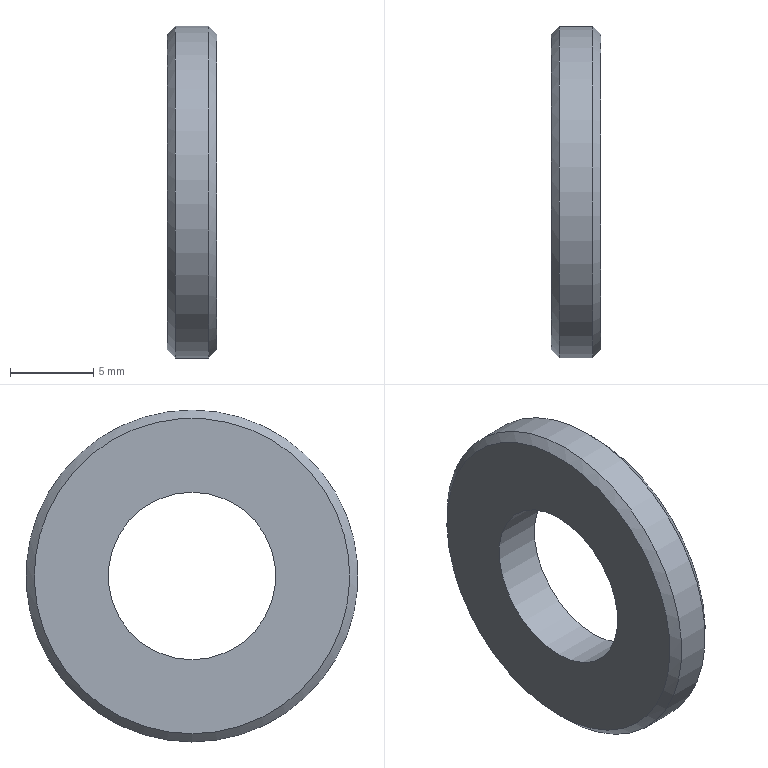Component | NX | 11_WASHER | 1 solid | 6 faces | box 3 x 20 x 20 mm | volume 687 mm3 | plane 2 | cylinder 2 | cone 2 | commonest cylinder face diameters 10.1 x1 20 x1
STEP:
#1=CARTESIAN_POINT('',(0.,0.,0.));
#2=DIRECTION('',(0.,0.,1.));
#3=DIRECTION('',(1.,0.,0.));
#4=AXIS2_PLACEMENT_3D('',#1,#2,#3);
#5=CARTESIAN_POINT('',(-0.,-0.,72.5));
#6=VERTEX_POINT('',#5);
#7=CARTESIAN_POINT('',(-0.,-0.,63.));
#8=DIRECTION('',(1.,0.,0.));
#9=DIRECTION('',(0.,0.,1.));
#10=AXIS2_PLACEMENT_3D('',#7,#8,#9);
#11=CIRCLE('',#10,9.5);
#12=CARTESIAN_POINT('',(-0.,-0.,73.));
#13=DIRECTION('',(-1.,0.,0.));
#14=DIRECTION('',(0.,0.,1.));
#15=AXIS2_PLACEMENT_3D('',#12,#13,#14);
#16=PLANE('',#15);
#17=CARTESIAN_POINT('',(-0.5,0.));
#18=CARTESIAN_POINT('',(-0.5,-16.454));
#19=CARTESIAN_POINT('',(-14.75,-8.227));
#20=CARTESIAN_POINT('',(-29.,-0.));
#21=CARTESIAN_POINT('',(-14.75,8.227));
#22=CARTESIAN_POINT('',(-0.5,16.454));
#23=CARTESIAN_POINT('',(-0.5,0.));
#24=(BOUNDED_CURVE()B_SPLINE_CURVE(2,(#17,#18,#19,#20,#21,#22,#23),.UNSPECIFIED.,.T.,.F.)B_SPLINE_CURVE_WITH_KNOTS((1,2,2,2,2,1),(-2.094,0.,2.094,4.189,6.283,8.378),.UNSPECIFIED.)CURVE()GEOMETRIC_REPRESENTATION_ITEM()RATIONAL_B_SPLINE_CURVE((1.,0.5,1.,0.5,1.,0.5,1.))REPRESENTATION_ITEM(''));
#25=(GEOMETRIC_REPRESENTATION_CONTEXT(2)PARAMETRIC_REPRESENTATION_CONTEXT()REPRESENTATION_CONTEXT('',''));
#26=DEFINITIONAL_REPRESENTATION('',(#24),#25);
#27=PCURVE('',#16,#26);
#28=CARTESIAN_POINT('',(-0.,-0.,63.));
#29=DIRECTION('',(-1.,0.,0.));
#30=DIRECTION('',(0.,0.,1.));
#31=AXIS2_PLACEMENT_3D('',#28,#29,#30);
#32=CONICAL_SURFACE('',#31,9.5,0.7854);
#33=CARTESIAN_POINT('',(6.283,0.));
#34=DIRECTION('',(-1.,0.));
#35=VECTOR('',#34,1.);
#36=LINE('',#33,#35);
#37=(GEOMETRIC_REPRESENTATION_CONTEXT(2)PARAMETRIC_REPRESENTATION_CONTEXT()REPRESENTATION_CONTEXT('',''));
#38=DEFINITIONAL_REPRESENTATION('',(#36),#37);
#39=PCURVE('',#32,#38);
#40=SURFACE_CURVE('',#11,(#27,#39),.PCURVE_S1.);
#41=EDGE_CURVE('',#6,#6,#40,.T.);
#42=ORIENTED_EDGE('',*,*,#41,.T.);
#43=EDGE_LOOP('',(#42));
#44=FACE_BOUND('',#43,.T.);
#45=CARTESIAN_POINT('',(0.,-0.,57.95));
#46=VERTEX_POINT('',#45);
#47=CARTESIAN_POINT('',(0.,-0.,63.));
#48=DIRECTION('',(1.,0.,0.));
#49=DIRECTION('',(0.,0.,-1.));
#50=AXIS2_PLACEMENT_3D('',#47,#48,#49);
#51=CIRCLE('',#50,5.05);
#52=CARTESIAN_POINT('',(-15.05,0.));
#53=CARTESIAN_POINT('',(-15.05,8.747));
#54=CARTESIAN_POINT('',(-7.475,4.373));
#55=CARTESIAN_POINT('',(0.1,0.));
#56=CARTESIAN_POINT('',(-7.475,-4.373));
#57=CARTESIAN_POINT('',(-15.05,-8.747));
#58=CARTESIAN_POINT('',(-15.05,0.));
#59=(BOUNDED_CURVE()B_SPLINE_CURVE(2,(#52,#53,#54,#55,#56,#57,#58),.UNSPECIFIED.,.T.,.F.)B_SPLINE_CURVE_WITH_KNOTS((1,2,2,2,2,1),(-2.094,0.,2.094,4.189,6.283,8.378),.UNSPECIFIED.)CURVE()GEOMETRIC_REPRESENTATION_ITEM()RATIONAL_B_SPLINE_CURVE((1.,0.5,1.,0.5,1.,0.5,1.))REPRESENTATION_ITEM(''));
#60=(GEOMETRIC_REPRESENTATION_CONTEXT(2)PARAMETRIC_REPRESENTATION_CONTEXT()REPRESENTATION_CONTEXT('',''));
#61=DEFINITIONAL_REPRESENTATION('',(#59),#60);
#62=PCURVE('',#16,#61);
#63=CARTESIAN_POINT('',(0.,-0.,63.));
#64=DIRECTION('',(1.,0.,0.));
#65=DIRECTION('',(0.,0.,-1.));
#66=AXIS2_PLACEMENT_3D('',#63,#64,#65);
#67=CYLINDRICAL_SURFACE('',#66,5.05);
#68=CARTESIAN_POINT('',(0.,0.));
#69=DIRECTION('',(1.,0.));
#70=VECTOR('',#69,1.);
#71=LINE('',#68,#70);
#72=(GEOMETRIC_REPRESENTATION_CONTEXT(2)PARAMETRIC_REPRESENTATION_CONTEXT()REPRESENTATION_CONTEXT('',''));
#73=DEFINITIONAL_REPRESENTATION('',(#71),#72);
#74=PCURVE('',#67,#73);
#75=SURFACE_CURVE('',#51,(#62,#74),.PCURVE_S1.);
#76=EDGE_CURVE('',#46,#46,#75,.T.);
#77=ORIENTED_EDGE('',*,*,#76,.F.);
#78=EDGE_LOOP('',(#77));
#79=FACE_BOUND('',#78,.T.);
#80=ADVANCED_FACE('',(#44,#79),#16,.F.);
#81=CARTESIAN_POINT('',(-3.,-0.,57.95));
#82=VERTEX_POINT('',#81);
#83=CARTESIAN_POINT('',(-3.,-0.,63.));
#84=DIRECTION('',(1.,0.,0.));
#85=DIRECTION('',(0.,0.,-1.));
#86=AXIS2_PLACEMENT_3D('',#83,#84,#85);
#87=CIRCLE('',#86,5.05);
#88=CARTESIAN_POINT('',(0.,-3.));
#89=DIRECTION('',(1.,0.));
#90=VECTOR('',#89,1.);
#91=LINE('',#88,#90);
#92=(GEOMETRIC_REPRESENTATION_CONTEXT(2)PARAMETRIC_REPRESENTATION_CONTEXT()REPRESENTATION_CONTEXT('',''));
#93=DEFINITIONAL_REPRESENTATION('',(#91),#92);
#94=PCURVE('',#67,#93);
#95=CARTESIAN_POINT('',(-3.,-0.,68.05));
#96=DIRECTION('',(1.,0.,0.));
#97=DIRECTION('',(0.,0.,-1.));
#98=AXIS2_PLACEMENT_3D('',#95,#96,#97);
#99=PLANE('',#98);
#100=CARTESIAN_POINT('',(5.05,0.));
#101=DIRECTION('',(1.,0.));
#102=AXIS2_PLACEMENT_2D('',#100,#101);
#103=CIRCLE('',#102,5.05);
#104=(GEOMETRIC_REPRESENTATION_CONTEXT(2)PARAMETRIC_REPRESENTATION_CONTEXT()REPRESENTATION_CONTEXT('',''));
#105=DEFINITIONAL_REPRESENTATION('',(#103),#104);
#106=PCURVE('',#99,#105);
#107=SURFACE_CURVE('',#87,(#94,#106),.PCURVE_S1.);
#108=EDGE_CURVE('',#82,#82,#107,.T.);
#109=ORIENTED_EDGE('',*,*,#108,.T.);
#110=CARTESIAN_POINT('',(-3.,-0.,57.95));
#111=CARTESIAN_POINT('',(0.,-0.,57.95));
#112=B_SPLINE_CURVE_WITH_KNOTS('',1,(#110,#111),.UNSPECIFIED.,.F.,.F.,(2,2),(-3.,0.),.PIECEWISE_BEZIER_KNOTS.);
#113=CARTESIAN_POINT('',(6.283,0.));
#114=DIRECTION('',(0.,1.));
#115=VECTOR('',#114,1.);
#116=LINE('',#113,#115);
#117=(GEOMETRIC_REPRESENTATION_CONTEXT(2)PARAMETRIC_REPRESENTATION_CONTEXT()REPRESENTATION_CONTEXT('',''));
#118=DEFINITIONAL_REPRESENTATION('',(#116),#117);
#119=PCURVE('',#67,#118);
#120=CARTESIAN_POINT('',(0.,0.));
#121=DIRECTION('',(0.,1.));
#122=VECTOR('',#121,1.);
#123=LINE('',#120,#122);
#124=(GEOMETRIC_REPRESENTATION_CONTEXT(2)PARAMETRIC_REPRESENTATION_CONTEXT()REPRESENTATION_CONTEXT('',''));
#125=DEFINITIONAL_REPRESENTATION('',(#123),#124);
#126=PCURVE('',#67,#125);
#127=SEAM_CURVE('',#112,(#119,#126),.PCURVE_S1.);
#128=EDGE_CURVE('',#82,#46,#127,.T.);
#129=ORIENTED_EDGE('',*,*,#128,.T.);
#130=ORIENTED_EDGE('',*,*,#76,.F.);
#131=ORIENTED_EDGE('',*,*,#128,.F.);
#132=EDGE_LOOP('',(#109,#129,#130,#131));
#133=FACE_BOUND('',#132,.F.);
#134=ADVANCED_FACE('',(#133),#67,.F.);
#135=CARTESIAN_POINT('',(-3.,-0.,53.5));
#136=VERTEX_POINT('',#135);
#137=CARTESIAN_POINT('',(-3.,-0.,63.));
#138=DIRECTION('',(-1.,0.,0.));
#139=DIRECTION('',(0.,0.,-1.));
#140=AXIS2_PLACEMENT_3D('',#137,#138,#139);
#141=CIRCLE('',#140,9.5);
#142=CARTESIAN_POINT('',(14.55,0.));
#143=CARTESIAN_POINT('',(14.55,-16.454));
#144=CARTESIAN_POINT('',(0.3,-8.227));
#145=CARTESIAN_POINT('',(-13.95,-0.));
#146=CARTESIAN_POINT('',(0.3,8.227));
#147=CARTESIAN_POINT('',(14.55,16.454));
#148=CARTESIAN_POINT('',(14.55,0.));
#149=(BOUNDED_CURVE()B_SPLINE_CURVE(2,(#142,#143,#144,#145,#146,#147,#148),.UNSPECIFIED.,.T.,.F.)B_SPLINE_CURVE_WITH_KNOTS((1,2,2,2,2,1),(-2.094,0.,2.094,4.189,6.283,8.378),.UNSPECIFIED.)CURVE()GEOMETRIC_REPRESENTATION_ITEM()RATIONAL_B_SPLINE_CURVE((1.,0.5,1.,0.5,1.,0.5,1.))REPRESENTATION_ITEM(''));
#150=(GEOMETRIC_REPRESENTATION_CONTEXT(2)PARAMETRIC_REPRESENTATION_CONTEXT()REPRESENTATION_CONTEXT('',''));
#151=DEFINITIONAL_REPRESENTATION('',(#149),#150);
#152=PCURVE('',#99,#151);
#153=CARTESIAN_POINT('',(-2.5,-0.,63.));
#154=DIRECTION('',(1.,0.,0.));
#155=DIRECTION('',(0.,0.,-1.));
#156=AXIS2_PLACEMENT_3D('',#153,#154,#155);
#157=CONICAL_SURFACE('',#156,10.,0.7854);
#158=CARTESIAN_POINT('',(6.283,-0.5));
#159=DIRECTION('',(-1.,0.));
#160=VECTOR('',#159,1.);
#161=LINE('',#158,#160);
#162=(GEOMETRIC_REPRESENTATION_CONTEXT(2)PARAMETRIC_REPRESENTATION_CONTEXT()REPRESENTATION_CONTEXT('',''));
#163=DEFINITIONAL_REPRESENTATION('',(#161),#162);
#164=PCURVE('',#157,#163);
#165=SURFACE_CURVE('',#141,(#152,#164),.PCURVE_S1.);
#166=EDGE_CURVE('',#136,#136,#165,.T.);
#167=ORIENTED_EDGE('',*,*,#166,.T.);
#168=EDGE_LOOP('',(#167));
#169=FACE_BOUND('',#168,.T.);
#170=ORIENTED_EDGE('',*,*,#108,.T.);
#171=EDGE_LOOP('',(#170));
#172=FACE_BOUND('',#171,.T.);
#173=ADVANCED_FACE('',(#169,#172),#99,.F.);
#174=CARTESIAN_POINT('',(-2.5,-0.,53.));
#175=VERTEX_POINT('',#174);
#176=CARTESIAN_POINT('',(-2.5,-0.,63.));
#177=DIRECTION('',(1.,0.,0.));
#178=DIRECTION('',(0.,0.,-1.));
#179=AXIS2_PLACEMENT_3D('',#176,#177,#178);
#180=CIRCLE('',#179,10.);
#181=CARTESIAN_POINT('',(0.,-0.,63.));
#182=DIRECTION('',(1.,0.,0.));
#183=DIRECTION('',(0.,0.,-1.));
#184=AXIS2_PLACEMENT_3D('',#181,#182,#183);
#185=CYLINDRICAL_SURFACE('',#184,10.);
#186=CARTESIAN_POINT('',(0.,-2.5));
#187=DIRECTION('',(1.,0.));
#188=VECTOR('',#187,1.);
#189=LINE('',#186,#188);
#190=(GEOMETRIC_REPRESENTATION_CONTEXT(2)PARAMETRIC_REPRESENTATION_CONTEXT()REPRESENTATION_CONTEXT('',''));
#191=DEFINITIONAL_REPRESENTATION('',(#189),#190);
#192=PCURVE('',#185,#191);
#193=CARTESIAN_POINT('',(0.,0.));
#194=DIRECTION('',(1.,0.));
#195=VECTOR('',#194,1.);
#196=LINE('',#193,#195);
#197=(GEOMETRIC_REPRESENTATION_CONTEXT(2)PARAMETRIC_REPRESENTATION_CONTEXT()REPRESENTATION_CONTEXT('',''));
#198=DEFINITIONAL_REPRESENTATION('',(#196),#197);
#199=PCURVE('',#157,#198);
#200=SURFACE_CURVE('',#180,(#192,#199),.PCURVE_S1.);
#201=EDGE_CURVE('',#175,#175,#200,.T.);
#202=ORIENTED_EDGE('',*,*,#201,.T.);
#203=CARTESIAN_POINT('',(-0.5,-0.,53.));
#204=VERTEX_POINT('',#203);
#205=CARTESIAN_POINT('',(-2.5,-0.,53.));
#206=CARTESIAN_POINT('',(-0.5,-0.,53.));
#207=B_SPLINE_CURVE_WITH_KNOTS('',1,(#205,#206),.UNSPECIFIED.,.F.,.F.,(2,2),(-2.5,-0.5),.PIECEWISE_BEZIER_KNOTS.);
#208=CARTESIAN_POINT('',(6.283,0.));
#209=DIRECTION('',(0.,1.));
#210=VECTOR('',#209,1.);
#211=LINE('',#208,#210);
#212=(GEOMETRIC_REPRESENTATION_CONTEXT(2)PARAMETRIC_REPRESENTATION_CONTEXT()REPRESENTATION_CONTEXT('',''));
#213=DEFINITIONAL_REPRESENTATION('',(#211),#212);
#214=PCURVE('',#185,#213);
#215=CARTESIAN_POINT('',(0.,0.));
#216=DIRECTION('',(0.,1.));
#217=VECTOR('',#216,1.);
#218=LINE('',#215,#217);
#219=(GEOMETRIC_REPRESENTATION_CONTEXT(2)PARAMETRIC_REPRESENTATION_CONTEXT()REPRESENTATION_CONTEXT('',''));
#220=DEFINITIONAL_REPRESENTATION('',(#218),#219);
#221=PCURVE('',#185,#220);
#222=SEAM_CURVE('',#207,(#214,#221),.PCURVE_S1.);
#223=EDGE_CURVE('',#175,#204,#222,.T.);
#224=ORIENTED_EDGE('',*,*,#223,.T.);
#225=CARTESIAN_POINT('',(-0.5,-0.,73.));
#226=VERTEX_POINT('',#225);
#227=CARTESIAN_POINT('',(-0.5,-0.,63.));
#228=DIRECTION('',(-1.,0.,0.));
#229=DIRECTION('',(0.,0.,1.));
#230=AXIS2_PLACEMENT_3D('',#227,#228,#229);
#231=CIRCLE('',#230,10.);
#232=CARTESIAN_POINT('',(9.425,-0.5));
#233=DIRECTION('',(-1.,0.));
#234=VECTOR('',#233,1.);
#235=LINE('',#232,#234);
#236=(GEOMETRIC_REPRESENTATION_CONTEXT(2)PARAMETRIC_REPRESENTATION_CONTEXT()REPRESENTATION_CONTEXT('',''));
#237=DEFINITIONAL_REPRESENTATION('',(#235),#236);
#238=PCURVE('',#185,#237);
#239=CARTESIAN_POINT('',(0.,0.5));
#240=DIRECTION('',(1.,0.));
#241=VECTOR('',#240,1.);
#242=LINE('',#239,#241);
#243=(GEOMETRIC_REPRESENTATION_CONTEXT(2)PARAMETRIC_REPRESENTATION_CONTEXT()REPRESENTATION_CONTEXT('',''));
#244=DEFINITIONAL_REPRESENTATION('',(#242),#243);
#245=PCURVE('',#32,#244);
#246=SURFACE_CURVE('',#231,(#238,#245),.PCURVE_S1.);
#247=EDGE_CURVE('',#204,#226,#246,.T.);
#248=ORIENTED_EDGE('',*,*,#247,.T.);
#249=CARTESIAN_POINT('',(-0.5,-0.,63.));
#250=DIRECTION('',(-1.,0.,0.));
#251=DIRECTION('',(0.,0.,1.));
#252=AXIS2_PLACEMENT_3D('',#249,#250,#251);
#253=CIRCLE('',#252,10.);
#254=CARTESIAN_POINT('',(3.142,-0.5));
#255=DIRECTION('',(-1.,0.));
#256=VECTOR('',#255,1.);
#257=LINE('',#254,#256);
#258=(GEOMETRIC_REPRESENTATION_CONTEXT(2)PARAMETRIC_REPRESENTATION_CONTEXT()REPRESENTATION_CONTEXT('',''));
#259=DEFINITIONAL_REPRESENTATION('',(#257),#258);
#260=PCURVE('',#185,#259);
#261=CARTESIAN_POINT('',(0.,0.5));
#262=DIRECTION('',(1.,0.));
#263=VECTOR('',#262,1.);
#264=LINE('',#261,#263);
#265=(GEOMETRIC_REPRESENTATION_CONTEXT(2)PARAMETRIC_REPRESENTATION_CONTEXT()REPRESENTATION_CONTEXT('',''));
#266=DEFINITIONAL_REPRESENTATION('',(#264),#265);
#267=PCURVE('',#32,#266);
#268=SURFACE_CURVE('',#253,(#260,#267),.PCURVE_S1.);
#269=EDGE_CURVE('',#226,#204,#268,.T.);
#270=ORIENTED_EDGE('',*,*,#269,.T.);
#271=ORIENTED_EDGE('',*,*,#223,.F.);
#272=EDGE_LOOP('',(#202,#224,#248,#270,#271));
#273=FACE_BOUND('',#272,.T.);
#274=ADVANCED_FACE('',(#273),#185,.T.);
#275=ORIENTED_EDGE('',*,*,#166,.F.);
#276=CARTESIAN_POINT('',(-3.,-0.,53.5));
#277=CARTESIAN_POINT('',(-2.5,-0.,53.));
#278=B_SPLINE_CURVE_WITH_KNOTS('',1,(#276,#277),.UNSPECIFIED.,.F.,.F.,(2,2),(-0.7071,0.),.PIECEWISE_BEZIER_KNOTS.);
#279=CARTESIAN_POINT('',(6.283,0.));
#280=DIRECTION('',(0.,1.));
#281=VECTOR('',#280,1.);
#282=LINE('',#279,#281);
#283=(GEOMETRIC_REPRESENTATION_CONTEXT(2)PARAMETRIC_REPRESENTATION_CONTEXT()REPRESENTATION_CONTEXT('',''));
#284=DEFINITIONAL_REPRESENTATION('',(#282),#283);
#285=PCURVE('',#157,#284);
#286=CARTESIAN_POINT('',(0.,0.));
#287=DIRECTION('',(0.,1.));
#288=VECTOR('',#287,1.);
#289=LINE('',#286,#288);
#290=(GEOMETRIC_REPRESENTATION_CONTEXT(2)PARAMETRIC_REPRESENTATION_CONTEXT()REPRESENTATION_CONTEXT('',''));
#291=DEFINITIONAL_REPRESENTATION('',(#289),#290);
#292=PCURVE('',#157,#291);
#293=SEAM_CURVE('',#278,(#285,#292),.PCURVE_S1.);
#294=EDGE_CURVE('',#136,#175,#293,.T.);
#295=ORIENTED_EDGE('',*,*,#294,.T.);
#296=ORIENTED_EDGE('',*,*,#201,.F.);
#297=ORIENTED_EDGE('',*,*,#294,.F.);
#298=EDGE_LOOP('',(#275,#295,#296,#297));
#299=FACE_BOUND('',#298,.T.);
#300=ADVANCED_FACE('',(#299),#157,.T.);
#301=ORIENTED_EDGE('',*,*,#269,.F.);
#302=CARTESIAN_POINT('',(-0.,-0.,72.5));
#303=CARTESIAN_POINT('',(-0.5,-0.,73.));
#304=B_SPLINE_CURVE_WITH_KNOTS('',1,(#302,#303),.UNSPECIFIED.,.F.,.F.,(2,2),(0.,0.7071),.PIECEWISE_BEZIER_KNOTS.);
#305=CARTESIAN_POINT('',(0.,0.));
#306=DIRECTION('',(0.,1.));
#307=VECTOR('',#306,1.);
#308=LINE('',#305,#307);
#309=(GEOMETRIC_REPRESENTATION_CONTEXT(2)PARAMETRIC_REPRESENTATION_CONTEXT()REPRESENTATION_CONTEXT('',''));
#310=DEFINITIONAL_REPRESENTATION('',(#308),#309);
#311=PCURVE('',#32,#310);
#312=CARTESIAN_POINT('',(6.283,0.));
#313=DIRECTION('',(0.,1.));
#314=VECTOR('',#313,1.);
#315=LINE('',#312,#314);
#316=(GEOMETRIC_REPRESENTATION_CONTEXT(2)PARAMETRIC_REPRESENTATION_CONTEXT()REPRESENTATION_CONTEXT('',''));
#317=DEFINITIONAL_REPRESENTATION('',(#315),#316);
#318=PCURVE('',#32,#317);
#319=SEAM_CURVE('',#304,(#311,#318),.PCURVE_S1.);
#320=EDGE_CURVE('',#6,#226,#319,.T.);
#321=ORIENTED_EDGE('',*,*,#320,.F.);
#322=ORIENTED_EDGE('',*,*,#41,.F.);
#323=ORIENTED_EDGE('',*,*,#320,.T.);
#324=ORIENTED_EDGE('',*,*,#247,.F.);
#325=EDGE_LOOP('',(#301,#321,#322,#323,#324));
#326=FACE_BOUND('',#325,.T.);
#327=ADVANCED_FACE('',(#326),#32,.T.);
#328=CLOSED_SHELL('',(#80,#134,#173,#274,#300,#327));
#329=MANIFOLD_SOLID_BREP('',#328);
#330=(LENGTH_UNIT()NAMED_UNIT(*)SI_UNIT(.MILLI.,.METRE.));
#331=UNCERTAINTY_MEASURE_WITH_UNIT(LENGTH_MEASURE(0.00001),#330,'','');
#332=(NAMED_UNIT(*)PLANE_ANGLE_UNIT()SI_UNIT($,.RADIAN.));
#333=(NAMED_UNIT(*)SI_UNIT($,.STERADIAN.)SOLID_ANGLE_UNIT());
#334=(GEOMETRIC_REPRESENTATION_CONTEXT(3)GLOBAL_UNCERTAINTY_ASSIGNED_CONTEXT((#331))GLOBAL_UNIT_ASSIGNED_CONTEXT((#330,#332,#333))REPRESENTATION_CONTEXT('',''));
#335=ADVANCED_BREP_SHAPE_REPRESENTATION('',(#4,#329),#334);